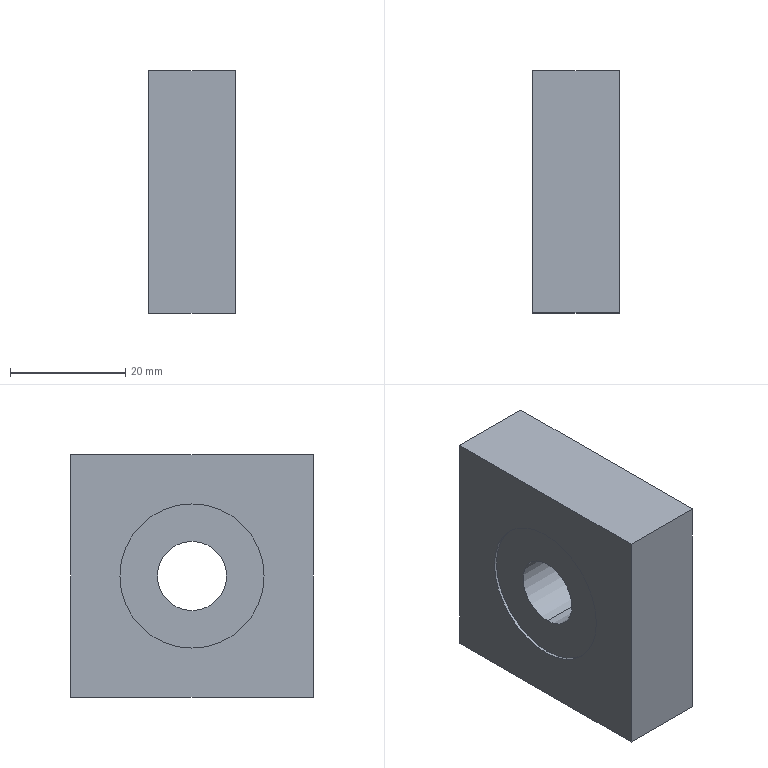Component | SolidWorks | NutFlatWasher-1 | 1 solid | 11 faces | box 15 x 42 x 42 mm | volume 24575 mm3 | plane 7 | cylinder 4 | commonest cylinder face diameters 25 x2 12 x2
build123d program:
from build123d import *

# Parameters (mm, degrees)
SKETCH1_2_W         = 42
SKETCH1_2_H         = 42
SKETCH1_2_R         = 6
BOSS_EXTRUDE1_DEPTH = 15
SKETCH1_R           = 12.5
BEARINGRELIEF_DEPTH = 0.5


with BuildPart() as part:
    # Sketch1_2 → Boss-Extrude1 (new body)
    with BuildSketch(Plane.XY):
        with Locations((21, 21)):
            Rectangle(SKETCH1_2_W, SKETCH1_2_H)
        with Locations((21, 21)):
            Circle(SKETCH1_2_R, mode=Mode.SUBTRACT)
    extrude(amount=BOSS_EXTRUDE1_DEPTH)

    # Sketch1 → BearingRelief (cut)
    with BuildSketch(Plane(origin=(0, 0, 0), x_dir=(-1, 0, 0), z_dir=(0, 0, -1))):
        with Locations((-21, 21)):
            Circle(SKETCH1_R)
    extrude(amount=-BEARINGRELIEF_DEPTH, mode=Mode.SUBTRACT)


solid = part.part

# Placed as in the assembly
solid = solid.moved(Location((-181.522, -1.055, 24.551), (0, 90, 0)))
STEP:
#1=COLOUR_RGB('',0.7922,0.8196,0.9333);
#2=FILL_AREA_STYLE_COLOUR('',#1);
#3=FILL_AREA_STYLE('',(#2));
#4=SURFACE_STYLE_FILL_AREA(#3);
#5=SURFACE_SIDE_STYLE('',(#4));
#6=SURFACE_STYLE_USAGE(.BOTH.,#5);
#7=PRESENTATION_STYLE_ASSIGNMENT((#6));
#8=CARTESIAN_POINT('',(-7.127,0.7853,-0.3523));
#9=VERTEX_POINT('',#8);
#10=CARTESIAN_POINT('',(-7.127,0.7853,0.6319));
#11=VERTEX_POINT('',#10);
#12=CARTESIAN_POINT('',(-7.127,0.7853,0.1398));
#13=DIRECTION('',(-1.,0.,0.));
#14=DIRECTION('',(0.,0.,1.));
#15=AXIS2_PLACEMENT_3D('',#12,#13,#14);
#16=CIRCLE('',#15,0.4921);
#17=EDGE_CURVE('',#9,#11,#16,.T.);
#18=ORIENTED_EDGE('',*,*,#17,.F.);
#19=CARTESIAN_POINT('',(-7.147,0.7853,-0.3523));
#20=VERTEX_POINT('',#19);
#21=CARTESIAN_POINT('',(-7.127,0.7853,-0.3523));
#22=DIRECTION('',(-1.,0.,0.));
#23=VECTOR('',#22,39.37);
#24=LINE('',#21,#23);
#25=EDGE_CURVE('',#9,#20,#24,.T.);
#26=ORIENTED_EDGE('',*,*,#25,.T.);
#27=CARTESIAN_POINT('',(-7.147,0.7853,0.6319));
#28=VERTEX_POINT('',#27);
#29=CARTESIAN_POINT('',(-7.147,0.7853,0.1398));
#30=DIRECTION('',(-1.,0.,0.));
#31=DIRECTION('',(0.,0.,1.));
#32=AXIS2_PLACEMENT_3D('',#29,#30,#31);
#33=CIRCLE('',#32,0.4921);
#34=EDGE_CURVE('',#20,#28,#33,.T.);
#35=ORIENTED_EDGE('',*,*,#34,.T.);
#36=CARTESIAN_POINT('',(-7.127,0.7853,0.6319));
#37=DIRECTION('',(-1.,0.,0.));
#38=VECTOR('',#37,39.37);
#39=LINE('',#36,#38);
#40=EDGE_CURVE('',#11,#28,#39,.T.);
#41=ORIENTED_EDGE('',*,*,#40,.F.);
#42=EDGE_LOOP('',(#18,#26,#35,#41));
#43=FACE_OUTER_BOUND('',#42,.T.);
#44=CARTESIAN_POINT('',(-7.127,0.7853,0.1398));
#45=DIRECTION('',(-1.,0.,0.));
#46=DIRECTION('',(0.,0.,1.));
#47=AXIS2_PLACEMENT_3D('',#44,#45,#46);
#48=CYLINDRICAL_SURFACE('',#47,0.4921);
#49=ADVANCED_FACE('',(#43),#48,.F.);
#50=CARTESIAN_POINT('',(-6.556,0.7853,0.376));
#51=VERTEX_POINT('',#50);
#52=CARTESIAN_POINT('',(-6.556,0.7853,-0.09643));
#53=VERTEX_POINT('',#52);
#54=CARTESIAN_POINT('',(-6.556,0.7853,0.1398));
#55=DIRECTION('',(1.,-0.,-0.));
#56=DIRECTION('',(0.,0.,-1.));
#57=AXIS2_PLACEMENT_3D('',#54,#55,#56);
#58=CIRCLE('',#57,0.2362);
#59=EDGE_CURVE('',#51,#53,#58,.T.);
#60=ORIENTED_EDGE('',*,*,#59,.T.);
#61=CARTESIAN_POINT('',(-7.127,0.7853,-0.09643));
#62=VERTEX_POINT('',#61);
#63=CARTESIAN_POINT('',(-6.556,0.7853,-0.09643));
#64=DIRECTION('',(-1.,0.,0.));
#65=VECTOR('',#64,39.37);
#66=LINE('',#63,#65);
#67=EDGE_CURVE('',#53,#62,#66,.T.);
#68=ORIENTED_EDGE('',*,*,#67,.T.);
#69=CARTESIAN_POINT('',(-7.127,0.7853,0.376));
#70=VERTEX_POINT('',#69);
#71=CARTESIAN_POINT('',(-7.127,0.7853,0.1398));
#72=DIRECTION('',(-1.,0.,0.));
#73=DIRECTION('',(0.,0.,1.));
#74=AXIS2_PLACEMENT_3D('',#71,#72,#73);
#75=CIRCLE('',#74,0.2362);
#76=EDGE_CURVE('',#62,#70,#75,.T.);
#77=ORIENTED_EDGE('',*,*,#76,.T.);
#78=CARTESIAN_POINT('',(-6.556,0.7853,0.376));
#79=DIRECTION('',(-1.,0.,0.));
#80=VECTOR('',#79,39.37);
#81=LINE('',#78,#80);
#82=EDGE_CURVE('',#51,#70,#81,.T.);
#83=ORIENTED_EDGE('',*,*,#82,.F.);
#84=EDGE_LOOP('',(#60,#68,#77,#83));
#85=FACE_OUTER_BOUND('',#84,.T.);
#86=CARTESIAN_POINT('',(-6.556,0.7853,0.1398));
#87=DIRECTION('',(-1.,0.,0.));
#88=DIRECTION('',(0.,0.,1.));
#89=AXIS2_PLACEMENT_3D('',#86,#87,#88);
#90=CYLINDRICAL_SURFACE('',#89,0.2362);
#91=ADVANCED_FACE('',(#85),#90,.F.);
#92=ORIENTED_EDGE('',*,*,#67,.F.);
#93=CARTESIAN_POINT('',(-6.556,0.7853,0.1398));
#94=DIRECTION('',(1.,-0.,-0.));
#95=DIRECTION('',(0.,0.,-1.));
#96=AXIS2_PLACEMENT_3D('',#93,#94,#95);
#97=CIRCLE('',#96,0.2362);
#98=EDGE_CURVE('',#53,#51,#97,.T.);
#99=ORIENTED_EDGE('',*,*,#98,.T.);
#100=ORIENTED_EDGE('',*,*,#82,.T.);
#101=CARTESIAN_POINT('',(-7.127,0.7853,0.1398));
#102=DIRECTION('',(-1.,0.,0.));
#103=DIRECTION('',(0.,0.,1.));
#104=AXIS2_PLACEMENT_3D('',#101,#102,#103);
#105=CIRCLE('',#104,0.2362);
#106=EDGE_CURVE('',#70,#62,#105,.T.);
#107=ORIENTED_EDGE('',*,*,#106,.T.);
#108=EDGE_LOOP('',(#92,#99,#100,#107));
#109=FACE_OUTER_BOUND('',#108,.T.);
#110=CARTESIAN_POINT('',(-6.556,0.7853,0.1398));
#111=DIRECTION('',(-1.,0.,0.));
#112=DIRECTION('',(0.,0.,1.));
#113=AXIS2_PLACEMENT_3D('',#110,#111,#112);
#114=CYLINDRICAL_SURFACE('',#113,0.2362);
#115=ADVANCED_FACE('',(#109),#114,.F.);
#116=CARTESIAN_POINT('',(-6.556,1.612,0.9666));
#117=VERTEX_POINT('',#116);
#118=CARTESIAN_POINT('',(-6.556,-0.04152,0.9666));
#119=VERTEX_POINT('',#118);
#120=CARTESIAN_POINT('',(-6.556,-0.04152,0.9666));
#121=DIRECTION('',(-0.,-1.,0.));
#122=VECTOR('',#121,39.37);
#123=LINE('',#120,#122);
#124=EDGE_CURVE('',#117,#119,#123,.T.);
#125=ORIENTED_EDGE('',*,*,#124,.T.);
#126=CARTESIAN_POINT('',(-6.556,-0.04152,-0.687));
#127=VERTEX_POINT('',#126);
#128=CARTESIAN_POINT('',(-6.556,-0.04152,0.9666));
#129=DIRECTION('',(-0.,-0.,-1.));
#130=VECTOR('',#129,39.37);
#131=LINE('',#128,#130);
#132=EDGE_CURVE('',#119,#127,#131,.T.);
#133=ORIENTED_EDGE('',*,*,#132,.T.);
#134=CARTESIAN_POINT('',(-6.556,1.612,-0.687));
#135=VERTEX_POINT('',#134);
#136=CARTESIAN_POINT('',(-6.556,-0.04152,-0.687));
#137=DIRECTION('',(0.,1.,-0.));
#138=VECTOR('',#137,39.37);
#139=LINE('',#136,#138);
#140=EDGE_CURVE('',#127,#135,#139,.T.);
#141=ORIENTED_EDGE('',*,*,#140,.T.);
#142=CARTESIAN_POINT('',(-6.556,1.612,0.9666));
#143=DIRECTION('',(0.,0.,1.));
#144=VECTOR('',#143,39.37);
#145=LINE('',#142,#144);
#146=EDGE_CURVE('',#135,#117,#145,.T.);
#147=ORIENTED_EDGE('',*,*,#146,.T.);
#148=EDGE_LOOP('',(#125,#133,#141,#147));
#149=FACE_OUTER_BOUND('',#148,.T.);
#150=ORIENTED_EDGE('',*,*,#59,.F.);
#151=ORIENTED_EDGE('',*,*,#98,.F.);
#152=EDGE_LOOP('',(#150,#151));
#153=FACE_BOUND('',#152,.T.);
#154=CARTESIAN_POINT('',(-6.556,-0.04152,0.9666));
#155=DIRECTION('',(-1.,0.,0.));
#156=DIRECTION('',(0.,0.,1.));
#157=AXIS2_PLACEMENT_3D('',#154,#155,#156);
#158=PLANE('',#157);
#159=ADVANCED_FACE('',(#149,#153),#158,.F.);
#160=CARTESIAN_POINT('',(-7.147,0.7853,0.1398));
#161=DIRECTION('',(-1.,0.,0.));
#162=DIRECTION('',(0.,0.,1.));
#163=AXIS2_PLACEMENT_3D('',#160,#161,#162);
#164=CIRCLE('',#163,0.4921);
#165=EDGE_CURVE('',#28,#20,#164,.T.);
#166=ORIENTED_EDGE('',*,*,#165,.F.);
#167=ORIENTED_EDGE('',*,*,#34,.F.);
#168=EDGE_LOOP('',(#166,#167));
#169=FACE_BOUND('',#168,.T.);
#170=CARTESIAN_POINT('',(-7.147,1.612,0.9666));
#171=VERTEX_POINT('',#170);
#172=CARTESIAN_POINT('',(-7.147,-0.04152,0.9666));
#173=VERTEX_POINT('',#172);
#174=CARTESIAN_POINT('',(-7.147,-0.04152,0.9666));
#175=DIRECTION('',(-0.,-1.,0.));
#176=VECTOR('',#175,39.37);
#177=LINE('',#174,#176);
#178=EDGE_CURVE('',#171,#173,#177,.T.);
#179=ORIENTED_EDGE('',*,*,#178,.F.);
#180=CARTESIAN_POINT('',(-7.147,1.612,-0.687));
#181=VERTEX_POINT('',#180);
#182=CARTESIAN_POINT('',(-7.147,1.612,0.9666));
#183=DIRECTION('',(0.,0.,1.));
#184=VECTOR('',#183,39.37);
#185=LINE('',#182,#184);
#186=EDGE_CURVE('',#181,#171,#185,.T.);
#187=ORIENTED_EDGE('',*,*,#186,.F.);
#188=CARTESIAN_POINT('',(-7.147,-0.04152,-0.687));
#189=VERTEX_POINT('',#188);
#190=CARTESIAN_POINT('',(-7.147,-0.04152,-0.687));
#191=DIRECTION('',(0.,1.,-0.));
#192=VECTOR('',#191,39.37);
#193=LINE('',#190,#192);
#194=EDGE_CURVE('',#189,#181,#193,.T.);
#195=ORIENTED_EDGE('',*,*,#194,.F.);
#196=CARTESIAN_POINT('',(-7.147,-0.04152,0.9666));
#197=DIRECTION('',(-0.,-0.,-1.));
#198=VECTOR('',#197,39.37);
#199=LINE('',#196,#198);
#200=EDGE_CURVE('',#173,#189,#199,.T.);
#201=ORIENTED_EDGE('',*,*,#200,.F.);
#202=EDGE_LOOP('',(#179,#187,#195,#201));
#203=FACE_OUTER_BOUND('',#202,.T.);
#204=CARTESIAN_POINT('',(-7.147,-0.04152,0.9666));
#205=DIRECTION('',(-1.,0.,0.));
#206=DIRECTION('',(0.,0.,1.));
#207=AXIS2_PLACEMENT_3D('',#204,#205,#206);
#208=PLANE('',#207);
#209=ADVANCED_FACE('',(#169,#203),#208,.T.);
#210=ORIENTED_EDGE('',*,*,#178,.T.);
#211=CARTESIAN_POINT('',(-6.556,-0.04152,0.9666));
#212=DIRECTION('',(-1.,0.,0.));
#213=VECTOR('',#212,39.37);
#214=LINE('',#211,#213);
#215=EDGE_CURVE('',#119,#173,#214,.T.);
#216=ORIENTED_EDGE('',*,*,#215,.F.);
#217=ORIENTED_EDGE('',*,*,#124,.F.);
#218=CARTESIAN_POINT('',(-6.556,1.612,0.9666));
#219=DIRECTION('',(-1.,0.,0.));
#220=VECTOR('',#219,39.37);
#221=LINE('',#218,#220);
#222=EDGE_CURVE('',#117,#171,#221,.T.);
#223=ORIENTED_EDGE('',*,*,#222,.T.);
#224=EDGE_LOOP('',(#210,#216,#217,#223));
#225=FACE_OUTER_BOUND('',#224,.T.);
#226=CARTESIAN_POINT('',(-6.556,-0.04152,0.9666));
#227=DIRECTION('',(-0.,-0.,-1.));
#228=DIRECTION('',(-1.,0.,0.));
#229=AXIS2_PLACEMENT_3D('',#226,#227,#228);
#230=PLANE('',#229);
#231=ADVANCED_FACE('',(#225),#230,.F.);
#232=ORIENTED_EDGE('',*,*,#200,.T.);
#233=CARTESIAN_POINT('',(-6.556,-0.04152,-0.687));
#234=DIRECTION('',(-1.,0.,0.));
#235=VECTOR('',#234,39.37);
#236=LINE('',#233,#235);
#237=EDGE_CURVE('',#127,#189,#236,.T.);
#238=ORIENTED_EDGE('',*,*,#237,.F.);
#239=ORIENTED_EDGE('',*,*,#132,.F.);
#240=ORIENTED_EDGE('',*,*,#215,.T.);
#241=EDGE_LOOP('',(#232,#238,#239,#240));
#242=FACE_OUTER_BOUND('',#241,.T.);
#243=CARTESIAN_POINT('',(-6.556,-0.04152,0.9666));
#244=DIRECTION('',(0.,1.,-0.));
#245=DIRECTION('',(1.,-0.,-0.));
#246=AXIS2_PLACEMENT_3D('',#243,#244,#245);
#247=PLANE('',#246);
#248=ADVANCED_FACE('',(#242),#247,.F.);
#249=ORIENTED_EDGE('',*,*,#194,.T.);
#250=CARTESIAN_POINT('',(-6.556,1.612,-0.687));
#251=DIRECTION('',(-1.,0.,0.));
#252=VECTOR('',#251,39.37);
#253=LINE('',#250,#252);
#254=EDGE_CURVE('',#135,#181,#253,.T.);
#255=ORIENTED_EDGE('',*,*,#254,.F.);
#256=ORIENTED_EDGE('',*,*,#140,.F.);
#257=ORIENTED_EDGE('',*,*,#237,.T.);
#258=EDGE_LOOP('',(#249,#255,#256,#257));
#259=FACE_OUTER_BOUND('',#258,.T.);
#260=CARTESIAN_POINT('',(-6.556,-0.04152,-0.687));
#261=DIRECTION('',(0.,0.,1.));
#262=DIRECTION('',(1.,-0.,-0.));
#263=AXIS2_PLACEMENT_3D('',#260,#261,#262);
#264=PLANE('',#263);
#265=ADVANCED_FACE('',(#259),#264,.F.);
#266=ORIENTED_EDGE('',*,*,#186,.T.);
#267=ORIENTED_EDGE('',*,*,#222,.F.);
#268=ORIENTED_EDGE('',*,*,#146,.F.);
#269=ORIENTED_EDGE('',*,*,#254,.T.);
#270=EDGE_LOOP('',(#266,#267,#268,#269));
#271=FACE_OUTER_BOUND('',#270,.T.);
#272=CARTESIAN_POINT('',(-6.556,1.612,0.9666));
#273=DIRECTION('',(-0.,-1.,0.));
#274=DIRECTION('',(-1.,0.,0.));
#275=AXIS2_PLACEMENT_3D('',#272,#273,#274);
#276=PLANE('',#275);
#277=ADVANCED_FACE('',(#271),#276,.F.);
#278=ORIENTED_EDGE('',*,*,#25,.F.);
#279=CARTESIAN_POINT('',(-7.127,0.7853,0.1398));
#280=DIRECTION('',(-1.,0.,0.));
#281=DIRECTION('',(0.,0.,1.));
#282=AXIS2_PLACEMENT_3D('',#279,#280,#281);
#283=CIRCLE('',#282,0.4921);
#284=EDGE_CURVE('',#11,#9,#283,.T.);
#285=ORIENTED_EDGE('',*,*,#284,.F.);
#286=ORIENTED_EDGE('',*,*,#40,.T.);
#287=ORIENTED_EDGE('',*,*,#165,.T.);
#288=EDGE_LOOP('',(#278,#285,#286,#287));
#289=FACE_OUTER_BOUND('',#288,.T.);
#290=CARTESIAN_POINT('',(-7.127,0.7853,0.1398));
#291=DIRECTION('',(-1.,0.,0.));
#292=DIRECTION('',(0.,0.,1.));
#293=AXIS2_PLACEMENT_3D('',#290,#291,#292);
#294=CYLINDRICAL_SURFACE('',#293,0.4921);
#295=ADVANCED_FACE('',(#289),#294,.F.);
#296=ORIENTED_EDGE('',*,*,#106,.F.);
#297=ORIENTED_EDGE('',*,*,#76,.F.);
#298=EDGE_LOOP('',(#296,#297));
#299=FACE_BOUND('',#298,.T.);
#300=ORIENTED_EDGE('',*,*,#284,.T.);
#301=ORIENTED_EDGE('',*,*,#17,.T.);
#302=EDGE_LOOP('',(#300,#301));
#303=FACE_OUTER_BOUND('',#302,.T.);
#304=CARTESIAN_POINT('',(-7.127,0.7853,0.1398));
#305=DIRECTION('',(-1.,0.,0.));
#306=DIRECTION('',(0.,0.,1.));
#307=AXIS2_PLACEMENT_3D('',#304,#305,#306);
#308=PLANE('',#307);
#309=ADVANCED_FACE('',(#299,#303),#308,.T.);
#310=CLOSED_SHELL('',(#49,#91,#115,#159,#209,#231,#248,#265,#277,#295,#309));
#311=MANIFOLD_SOLID_BREP('',#310);
#312=STYLED_ITEM('',(#7),#311);
#313=(LENGTH_UNIT()NAMED_UNIT(*)SI_UNIT($,.METRE.));
#314=LENGTH_MEASURE_WITH_UNIT(LENGTH_MEASURE(0.0254),#313);
#315=DIMENSIONAL_EXPONENTS(1.,0.,0.,0.,0.,0.,0.);
#316=(CONVERSION_BASED_UNIT('',#314)LENGTH_UNIT()NAMED_UNIT(#315));
#317=UNCERTAINTY_MEASURE_WITH_UNIT(LENGTH_MEASURE(0.00001),#316,'','');
#318=(NAMED_UNIT(*)PLANE_ANGLE_UNIT()SI_UNIT($,.RADIAN.));
#319=(NAMED_UNIT(*)SI_UNIT($,.STERADIAN.)SOLID_ANGLE_UNIT());
#320=(GEOMETRIC_REPRESENTATION_CONTEXT(3)GLOBAL_UNCERTAINTY_ASSIGNED_CONTEXT((#317))GLOBAL_UNIT_ASSIGNED_CONTEXT((#316,#318,#319))REPRESENTATION_CONTEXT('',''));
#321=MECHANICAL_DESIGN_GEOMETRIC_PRESENTATION_REPRESENTATION('',(#312),#320);
#322=PRESENTATION_LAYER_ASSIGNMENT('','',(#312));
#323=CARTESIAN_POINT('',(0.,0.,0.));
#324=DIRECTION('',(0.,0.,1.));
#325=DIRECTION('',(1.,0.,0.));
#326=AXIS2_PLACEMENT_3D('',#323,#324,#325);
#327=(LENGTH_UNIT()NAMED_UNIT(*)SI_UNIT($,.METRE.));
#328=LENGTH_MEASURE_WITH_UNIT(LENGTH_MEASURE(0.0254),#327);
#329=DIMENSIONAL_EXPONENTS(1.,0.,0.,0.,0.,0.,0.);
#330=(CONVERSION_BASED_UNIT('',#328)LENGTH_UNIT()NAMED_UNIT(#329));
#331=UNCERTAINTY_MEASURE_WITH_UNIT(LENGTH_MEASURE(0.00001),#330,'','');
#332=(NAMED_UNIT(*)PLANE_ANGLE_UNIT()SI_UNIT($,.RADIAN.));
#333=(NAMED_UNIT(*)SI_UNIT($,.STERADIAN.)SOLID_ANGLE_UNIT());
#334=(GEOMETRIC_REPRESENTATION_CONTEXT(3)GLOBAL_UNCERTAINTY_ASSIGNED_CONTEXT((#331))GLOBAL_UNIT_ASSIGNED_CONTEXT((#330,#332,#333))REPRESENTATION_CONTEXT('',''));
#335=ADVANCED_BREP_SHAPE_REPRESENTATION('',(#311,#326),#334);